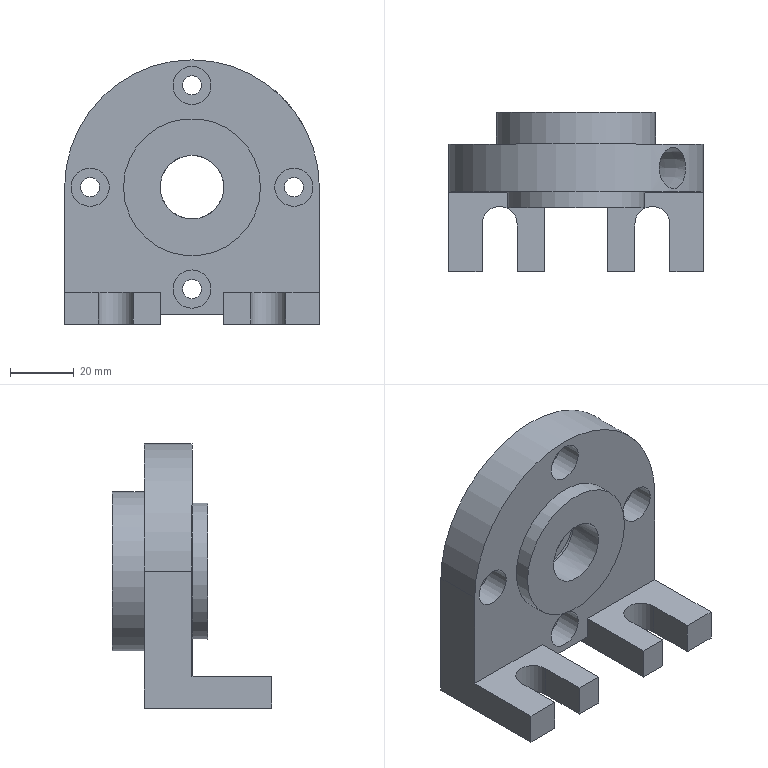Component | NX | FRONT_COVER | 1 solid | 47 faces | volume 108532 mm3 | plane 27 | cylinder 18 | cone 2 | commonest cylinder face diameters 6 x4 12 x4 20 x2 11 x2 11.5 x1 80 x1 43.052 x1 50 x1